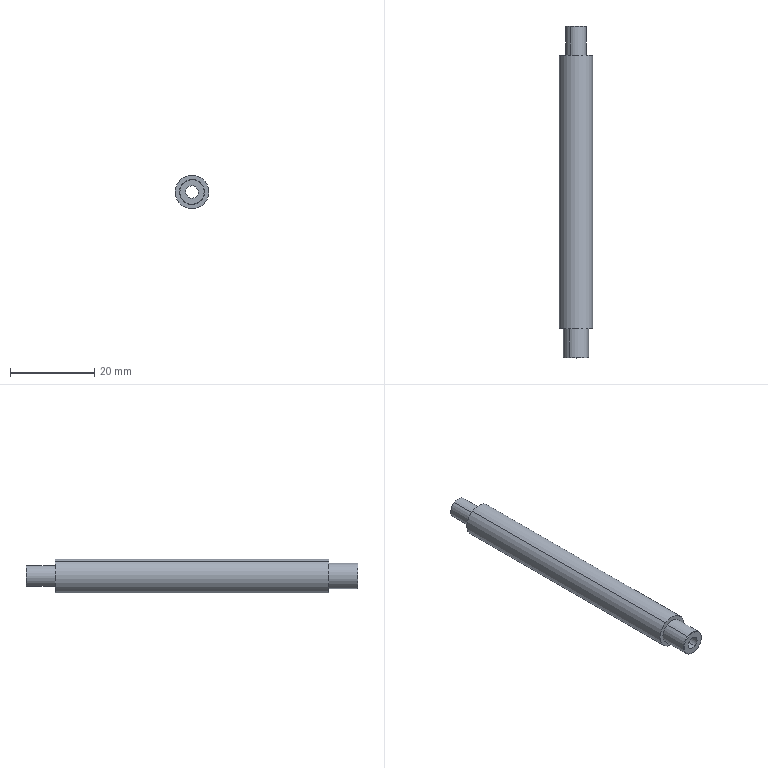Component | SolidWorks | WireFeedingTube-1 | 1 solid | 16 faces | box 8 x 79 x 8 mm | volume 3044 mm3 | cylinder 8 | cone 4 | plane 4 | commonest cylinder face diameters 6 x2 8 x2 5 x2 3 x2
build123d program:
from build123d import *

# Parameters (mm, degrees)
CHAMFER1_SIZE = 0.1


with BuildPart() as part:
    # Sketch1 → Revolve1 (revolve)
    with BuildSketch(Plane(origin=(0, 0, 0), x_dir=(0, 0, -1), z_dir=(1, 0, 0)), mode=Mode.PRIVATE) as revolve1_sk:
        Polygon((-13.875, 1.5), (65.125, 1.5), (65.125, 2.5), (58.125, 2.5), (58.125, 4), (-6.875, 4), (-6.875, 3), (-13.875, 3), align=None)
    revolve(revolve1_sk.sketch.rotate(Axis((0, 0, 14.85), (0, 0, -1)), 90), axis=Axis((0, 0, 14.85), (0, 0, -1)))

    # Chamfer1
    chamfer1_edges = [part.edges().sort_by_distance(p)[0] for p in [
        (-3, 0, 13.875),
        (-2.5, 0, -65.125),
    ]]
    chamfer(chamfer1_edges, length=CHAMFER1_SIZE)


solid = part.part

# Placed as in the assembly
solid = solid.moved(Location((37.32, 27.381, 185), (90, 0, 0)))
STEP:
#1=CARTESIAN_POINT('',(1.419,3.642,7.363));
#2=VERTEX_POINT('',#1);
#3=CARTESIAN_POINT('',(1.52,3.642,7.204));
#4=VERTEX_POINT('',#3);
#5=CARTESIAN_POINT('',(1.469,3.642,7.283));
#6=DIRECTION('',(0.,1.,-0.));
#7=DIRECTION('',(0.5343,0.,-0.8453));
#8=AXIS2_PLACEMENT_3D('',#5,#6,#7);
#9=CIRCLE('',#8,0.09449);
#10=EDGE_CURVE('',#2,#4,#9,.T.);
#11=ORIENTED_EDGE('',*,*,#10,.F.);
#12=CARTESIAN_POINT('',(1.417,3.638,7.367));
#13=VERTEX_POINT('',#12);
#14=CARTESIAN_POINT('',(1.417,3.638,7.367));
#15=DIRECTION('',(-0.3778,-0.7071,0.5977));
#16=VECTOR('',#15,39.37);
#17=LINE('',#14,#16);
#18=EDGE_CURVE('',#2,#13,#17,.T.);
#19=ORIENTED_EDGE('',*,*,#18,.T.);
#20=CARTESIAN_POINT('',(1.522,3.638,7.2));
#21=VERTEX_POINT('',#20);
#22=CARTESIAN_POINT('',(1.469,3.638,7.283));
#23=DIRECTION('',(-0.,-1.,0.));
#24=DIRECTION('',(0.5343,0.,-0.8453));
#25=AXIS2_PLACEMENT_3D('',#22,#23,#24);
#26=CIRCLE('',#25,0.09843);
#27=EDGE_CURVE('',#21,#13,#26,.T.);
#28=ORIENTED_EDGE('',*,*,#27,.F.);
#29=CARTESIAN_POINT('',(1.522,3.638,7.2));
#30=DIRECTION('',(0.3778,-0.7071,-0.5977));
#31=VECTOR('',#30,39.37);
#32=LINE('',#29,#31);
#33=EDGE_CURVE('',#4,#21,#32,.T.);
#34=ORIENTED_EDGE('',*,*,#33,.F.);
#35=EDGE_LOOP('',(#11,#19,#28,#34));
#36=FACE_OUTER_BOUND('',#35,.T.);
#37=CARTESIAN_POINT('',(1.469,3.638,7.283));
#38=DIRECTION('',(-0.,-1.,0.));
#39=DIRECTION('',(0.5343,0.,-0.8453));
#40=AXIS2_PLACEMENT_3D('',#37,#38,#39);
#41=CONICAL_SURFACE('',#40,0.09843,0.7854);
#42=ADVANCED_FACE('',(#36),#41,.T.);
#43=CARTESIAN_POINT('',(1.53,0.5317,7.187));
#44=VERTEX_POINT('',#43);
#45=CARTESIAN_POINT('',(1.408,0.5317,7.38));
#46=VERTEX_POINT('',#45);
#47=CARTESIAN_POINT('',(1.469,0.5317,7.283));
#48=DIRECTION('',(-0.,-1.,0.));
#49=DIRECTION('',(-0.5343,0.,0.8453));
#50=AXIS2_PLACEMENT_3D('',#47,#48,#49);
#51=CIRCLE('',#50,0.1142);
#52=EDGE_CURVE('',#44,#46,#51,.T.);
#53=ORIENTED_EDGE('',*,*,#52,.F.);
#54=CARTESIAN_POINT('',(1.532,0.5357,7.184));
#55=VERTEX_POINT('',#54);
#56=CARTESIAN_POINT('',(1.53,0.5317,7.187));
#57=DIRECTION('',(0.3778,0.7071,-0.5977));
#58=VECTOR('',#57,39.37);
#59=LINE('',#56,#58);
#60=EDGE_CURVE('',#44,#55,#59,.T.);
#61=ORIENTED_EDGE('',*,*,#60,.T.);
#62=CARTESIAN_POINT('',(1.406,0.5357,7.383));
#63=VERTEX_POINT('',#62);
#64=CARTESIAN_POINT('',(1.469,0.5357,7.283));
#65=DIRECTION('',(0.,1.,-0.));
#66=DIRECTION('',(-0.5343,0.,0.8453));
#67=AXIS2_PLACEMENT_3D('',#64,#65,#66);
#68=CIRCLE('',#67,0.1181);
#69=EDGE_CURVE('',#63,#55,#68,.T.);
#70=ORIENTED_EDGE('',*,*,#69,.F.);
#71=CARTESIAN_POINT('',(1.408,0.5317,7.38));
#72=DIRECTION('',(-0.3778,0.7071,0.5977));
#73=VECTOR('',#72,39.37);
#74=LINE('',#71,#73);
#75=EDGE_CURVE('',#46,#63,#74,.T.);
#76=ORIENTED_EDGE('',*,*,#75,.F.);
#77=EDGE_LOOP('',(#53,#61,#70,#76));
#78=FACE_OUTER_BOUND('',#77,.T.);
#79=CARTESIAN_POINT('',(1.469,0.5317,7.283));
#80=DIRECTION('',(0.,1.,-0.));
#81=DIRECTION('',(-0.5343,0.,0.8453));
#82=AXIS2_PLACEMENT_3D('',#79,#80,#81);
#83=CONICAL_SURFACE('',#82,0.1142,0.7854);
#84=ADVANCED_FACE('',(#78),#83,.T.);
#85=CARTESIAN_POINT('',(1.532,0.8073,7.184));
#86=VERTEX_POINT('',#85);
#87=CARTESIAN_POINT('',(1.406,0.8073,7.383));
#88=VERTEX_POINT('',#87);
#89=CARTESIAN_POINT('',(1.469,0.8073,7.283));
#90=DIRECTION('',(-0.,-1.,0.));
#91=DIRECTION('',(0.5343,0.,-0.8453));
#92=AXIS2_PLACEMENT_3D('',#89,#90,#91);
#93=CIRCLE('',#92,0.1181);
#94=EDGE_CURVE('',#86,#88,#93,.T.);
#95=ORIENTED_EDGE('',*,*,#94,.T.);
#96=CARTESIAN_POINT('',(1.406,0.4934,7.383));
#97=DIRECTION('',(-0.,-1.,0.));
#98=VECTOR('',#97,39.37);
#99=LINE('',#96,#98);
#100=EDGE_CURVE('',#88,#63,#99,.T.);
#101=ORIENTED_EDGE('',*,*,#100,.T.);
#102=ORIENTED_EDGE('',*,*,#69,.T.);
#103=CARTESIAN_POINT('',(1.532,0.4934,7.184));
#104=DIRECTION('',(-0.,-1.,0.));
#105=VECTOR('',#104,39.37);
#106=LINE('',#103,#105);
#107=EDGE_CURVE('',#86,#55,#106,.T.);
#108=ORIENTED_EDGE('',*,*,#107,.F.);
#109=EDGE_LOOP('',(#95,#101,#102,#108));
#110=FACE_OUTER_BOUND('',#109,.T.);
#111=CARTESIAN_POINT('',(1.469,0.4934,7.283));
#112=DIRECTION('',(-0.,-1.,0.));
#113=DIRECTION('',(0.5343,0.,-0.8453));
#114=AXIS2_PLACEMENT_3D('',#111,#112,#113);
#115=CYLINDRICAL_SURFACE('',#114,0.1181);
#116=ADVANCED_FACE('',(#110),#115,.T.);
#117=CARTESIAN_POINT('',(1.553,3.366,7.15));
#118=VERTEX_POINT('',#117);
#119=CARTESIAN_POINT('',(1.385,3.366,7.417));
#120=VERTEX_POINT('',#119);
#121=CARTESIAN_POINT('',(1.469,3.366,7.283));
#122=DIRECTION('',(-0.,-1.,0.));
#123=DIRECTION('',(0.5343,0.,-0.8453));
#124=AXIS2_PLACEMENT_3D('',#121,#122,#123);
#125=CIRCLE('',#124,0.1575);
#126=EDGE_CURVE('',#118,#120,#125,.T.);
#127=ORIENTED_EDGE('',*,*,#126,.T.);
#128=CARTESIAN_POINT('',(1.385,0.8073,7.417));
#129=VERTEX_POINT('',#128);
#130=CARTESIAN_POINT('',(1.385,0.4934,7.417));
#131=DIRECTION('',(-0.,-1.,0.));
#132=VECTOR('',#131,39.37);
#133=LINE('',#130,#132);
#134=EDGE_CURVE('',#120,#129,#133,.T.);
#135=ORIENTED_EDGE('',*,*,#134,.T.);
#136=CARTESIAN_POINT('',(1.553,0.8073,7.15));
#137=VERTEX_POINT('',#136);
#138=CARTESIAN_POINT('',(1.469,0.8073,7.283));
#139=DIRECTION('',(-0.,-1.,0.));
#140=DIRECTION('',(0.5343,0.,-0.8453));
#141=AXIS2_PLACEMENT_3D('',#138,#139,#140);
#142=CIRCLE('',#141,0.1575);
#143=EDGE_CURVE('',#137,#129,#142,.T.);
#144=ORIENTED_EDGE('',*,*,#143,.F.);
#145=CARTESIAN_POINT('',(1.553,0.4934,7.15));
#146=DIRECTION('',(-0.,-1.,0.));
#147=VECTOR('',#146,39.37);
#148=LINE('',#145,#147);
#149=EDGE_CURVE('',#118,#137,#148,.T.);
#150=ORIENTED_EDGE('',*,*,#149,.F.);
#151=EDGE_LOOP('',(#127,#135,#144,#150));
#152=FACE_OUTER_BOUND('',#151,.T.);
#153=CARTESIAN_POINT('',(1.469,0.4934,7.283));
#154=DIRECTION('',(-0.,-1.,0.));
#155=DIRECTION('',(0.5343,0.,-0.8453));
#156=AXIS2_PLACEMENT_3D('',#153,#154,#155);
#157=CYLINDRICAL_SURFACE('',#156,0.1575);
#158=ADVANCED_FACE('',(#152),#157,.T.);
#159=ORIENTED_EDGE('',*,*,#27,.T.);
#160=CARTESIAN_POINT('',(1.417,3.366,7.367));
#161=VERTEX_POINT('',#160);
#162=CARTESIAN_POINT('',(1.417,0.4934,7.367));
#163=DIRECTION('',(-0.,-1.,0.));
#164=VECTOR('',#163,39.37);
#165=LINE('',#162,#164);
#166=EDGE_CURVE('',#13,#161,#165,.T.);
#167=ORIENTED_EDGE('',*,*,#166,.T.);
#168=CARTESIAN_POINT('',(1.522,3.366,7.2));
#169=VERTEX_POINT('',#168);
#170=CARTESIAN_POINT('',(1.469,3.366,7.283));
#171=DIRECTION('',(-0.,-1.,0.));
#172=DIRECTION('',(0.5343,0.,-0.8453));
#173=AXIS2_PLACEMENT_3D('',#170,#171,#172);
#174=CIRCLE('',#173,0.09843);
#175=EDGE_CURVE('',#169,#161,#174,.T.);
#176=ORIENTED_EDGE('',*,*,#175,.F.);
#177=CARTESIAN_POINT('',(1.522,0.4934,7.2));
#178=DIRECTION('',(-0.,-1.,0.));
#179=VECTOR('',#178,39.37);
#180=LINE('',#177,#179);
#181=EDGE_CURVE('',#21,#169,#180,.T.);
#182=ORIENTED_EDGE('',*,*,#181,.F.);
#183=EDGE_LOOP('',(#159,#167,#176,#182));
#184=FACE_OUTER_BOUND('',#183,.T.);
#185=CARTESIAN_POINT('',(1.469,0.4934,7.283));
#186=DIRECTION('',(-0.,-1.,0.));
#187=DIRECTION('',(0.5343,0.,-0.8453));
#188=AXIS2_PLACEMENT_3D('',#185,#186,#187);
#189=CYLINDRICAL_SURFACE('',#188,0.09843);
#190=ADVANCED_FACE('',(#184),#189,.T.);
#191=CARTESIAN_POINT('',(1.438,3.642,7.333));
#192=VERTEX_POINT('',#191);
#193=CARTESIAN_POINT('',(1.501,3.642,7.234));
#194=VERTEX_POINT('',#193);
#195=CARTESIAN_POINT('',(1.469,3.642,7.283));
#196=DIRECTION('',(-0.,-1.,0.));
#197=DIRECTION('',(0.5343,0.,-0.8453));
#198=AXIS2_PLACEMENT_3D('',#195,#196,#197);
#199=CIRCLE('',#198,0.05906);
#200=EDGE_CURVE('',#192,#194,#199,.T.);
#201=ORIENTED_EDGE('',*,*,#200,.F.);
#202=CARTESIAN_POINT('',(1.438,0.5317,7.333));
#203=VERTEX_POINT('',#202);
#204=CARTESIAN_POINT('',(1.438,0.4934,7.333));
#205=DIRECTION('',(-0.,-1.,0.));
#206=VECTOR('',#205,39.37);
#207=LINE('',#204,#206);
#208=EDGE_CURVE('',#192,#203,#207,.T.);
#209=ORIENTED_EDGE('',*,*,#208,.T.);
#210=CARTESIAN_POINT('',(1.501,0.5317,7.234));
#211=VERTEX_POINT('',#210);
#212=CARTESIAN_POINT('',(1.469,0.5317,7.283));
#213=DIRECTION('',(-0.,-1.,0.));
#214=DIRECTION('',(0.5343,0.,-0.8453));
#215=AXIS2_PLACEMENT_3D('',#212,#213,#214);
#216=CIRCLE('',#215,0.05906);
#217=EDGE_CURVE('',#203,#211,#216,.T.);
#218=ORIENTED_EDGE('',*,*,#217,.T.);
#219=CARTESIAN_POINT('',(1.501,0.4934,7.234));
#220=DIRECTION('',(-0.,-1.,0.));
#221=VECTOR('',#220,39.37);
#222=LINE('',#219,#221);
#223=EDGE_CURVE('',#194,#211,#222,.T.);
#224=ORIENTED_EDGE('',*,*,#223,.F.);
#225=EDGE_LOOP('',(#201,#209,#218,#224));
#226=FACE_OUTER_BOUND('',#225,.T.);
#227=CARTESIAN_POINT('',(1.469,0.4934,7.283));
#228=DIRECTION('',(-0.,-1.,0.));
#229=DIRECTION('',(0.5343,0.,-0.8453));
#230=AXIS2_PLACEMENT_3D('',#227,#228,#229);
#231=CYLINDRICAL_SURFACE('',#230,0.05906);
#232=ADVANCED_FACE('',(#226),#231,.F.);
#233=CARTESIAN_POINT('',(1.469,0.5317,7.283));
#234=DIRECTION('',(-0.,-1.,0.));
#235=DIRECTION('',(-0.5343,0.,0.8453));
#236=AXIS2_PLACEMENT_3D('',#233,#234,#235);
#237=CIRCLE('',#236,0.1142);
#238=EDGE_CURVE('',#46,#44,#237,.T.);
#239=ORIENTED_EDGE('',*,*,#238,.T.);
#240=ORIENTED_EDGE('',*,*,#52,.T.);
#241=EDGE_LOOP('',(#239,#240));
#242=FACE_OUTER_BOUND('',#241,.T.);
#243=CARTESIAN_POINT('',(1.469,0.5317,7.283));
#244=DIRECTION('',(-0.,-1.,0.));
#245=DIRECTION('',(0.5343,0.,-0.8453));
#246=AXIS2_PLACEMENT_3D('',#243,#244,#245);
#247=CIRCLE('',#246,0.05906);
#248=EDGE_CURVE('',#211,#203,#247,.T.);
#249=ORIENTED_EDGE('',*,*,#248,.F.);
#250=ORIENTED_EDGE('',*,*,#217,.F.);
#251=EDGE_LOOP('',(#249,#250));
#252=FACE_BOUND('',#251,.T.);
#253=CARTESIAN_POINT('',(1.569,0.5317,7.347));
#254=DIRECTION('',(0.,1.,-0.));
#255=DIRECTION('',(-0.5343,0.,0.8453));
#256=AXIS2_PLACEMENT_3D('',#253,#254,#255);
#257=PLANE('',#256);
#258=ADVANCED_FACE('',(#242,#252),#257,.F.);
#259=ORIENTED_EDGE('',*,*,#208,.F.);
#260=CARTESIAN_POINT('',(1.469,3.642,7.283));
#261=DIRECTION('',(-0.,-1.,0.));
#262=DIRECTION('',(0.5343,0.,-0.8453));
#263=AXIS2_PLACEMENT_3D('',#260,#261,#262);
#264=CIRCLE('',#263,0.05906);
#265=EDGE_CURVE('',#194,#192,#264,.T.);
#266=ORIENTED_EDGE('',*,*,#265,.F.);
#267=ORIENTED_EDGE('',*,*,#223,.T.);
#268=ORIENTED_EDGE('',*,*,#248,.T.);
#269=EDGE_LOOP('',(#259,#266,#267,#268));
#270=FACE_OUTER_BOUND('',#269,.T.);
#271=CARTESIAN_POINT('',(1.469,0.4934,7.283));
#272=DIRECTION('',(-0.,-1.,0.));
#273=DIRECTION('',(0.5343,0.,-0.8453));
#274=AXIS2_PLACEMENT_3D('',#271,#272,#273);
#275=CYLINDRICAL_SURFACE('',#274,0.05906);
#276=ADVANCED_FACE('',(#270),#275,.F.);
#277=CARTESIAN_POINT('',(1.469,3.642,7.283));
#278=DIRECTION('',(0.,1.,-0.));
#279=DIRECTION('',(0.5343,0.,-0.8453));
#280=AXIS2_PLACEMENT_3D('',#277,#278,#279);
#281=CIRCLE('',#280,0.09449);
#282=EDGE_CURVE('',#4,#2,#281,.T.);
#283=ORIENTED_EDGE('',*,*,#282,.T.);
#284=ORIENTED_EDGE('',*,*,#10,.T.);
#285=EDGE_LOOP('',(#283,#284));
#286=FACE_OUTER_BOUND('',#285,.T.);
#287=ORIENTED_EDGE('',*,*,#265,.T.);
#288=ORIENTED_EDGE('',*,*,#200,.T.);
#289=EDGE_LOOP('',(#287,#288));
#290=FACE_BOUND('',#289,.T.);
#291=CARTESIAN_POINT('',(1.519,3.642,7.315));
#292=DIRECTION('',(-0.,-1.,0.));
#293=DIRECTION('',(0.5343,-0.,-0.8453));
#294=AXIS2_PLACEMENT_3D('',#291,#292,#293);
#295=PLANE('',#294);
#296=ADVANCED_FACE('',(#286,#290),#295,.F.);
#297=ORIENTED_EDGE('',*,*,#166,.F.);
#298=CARTESIAN_POINT('',(1.469,3.638,7.283));
#299=DIRECTION('',(-0.,-1.,0.));
#300=DIRECTION('',(0.5343,0.,-0.8453));
#301=AXIS2_PLACEMENT_3D('',#298,#299,#300);
#302=CIRCLE('',#301,0.09843);
#303=EDGE_CURVE('',#13,#21,#302,.T.);
#304=ORIENTED_EDGE('',*,*,#303,.T.);
#305=ORIENTED_EDGE('',*,*,#181,.T.);
#306=CARTESIAN_POINT('',(1.469,3.366,7.283));
#307=DIRECTION('',(-0.,-1.,0.));
#308=DIRECTION('',(0.5343,0.,-0.8453));
#309=AXIS2_PLACEMENT_3D('',#306,#307,#308);
#310=CIRCLE('',#309,0.09843);
#311=EDGE_CURVE('',#161,#169,#310,.T.);
#312=ORIENTED_EDGE('',*,*,#311,.F.);
#313=EDGE_LOOP('',(#297,#304,#305,#312));
#314=FACE_OUTER_BOUND('',#313,.T.);
#315=CARTESIAN_POINT('',(1.469,0.4934,7.283));
#316=DIRECTION('',(-0.,-1.,0.));
#317=DIRECTION('',(0.5343,0.,-0.8453));
#318=AXIS2_PLACEMENT_3D('',#315,#316,#317);
#319=CYLINDRICAL_SURFACE('',#318,0.09843);
#320=ADVANCED_FACE('',(#314),#319,.T.);
#321=ORIENTED_EDGE('',*,*,#126,.F.);
#322=CARTESIAN_POINT('',(1.469,3.366,7.283));
#323=DIRECTION('',(-0.,-1.,0.));
#324=DIRECTION('',(0.5343,0.,-0.8453));
#325=AXIS2_PLACEMENT_3D('',#322,#323,#324);
#326=CIRCLE('',#325,0.1575);
#327=EDGE_CURVE('',#120,#118,#326,.T.);
#328=ORIENTED_EDGE('',*,*,#327,.F.);
#329=EDGE_LOOP('',(#321,#328));
#330=FACE_OUTER_BOUND('',#329,.T.);
#331=ORIENTED_EDGE('',*,*,#175,.T.);
#332=ORIENTED_EDGE('',*,*,#311,.T.);
#333=EDGE_LOOP('',(#331,#332));
#334=FACE_BOUND('',#333,.T.);
#335=CARTESIAN_POINT('',(1.553,3.366,7.336));
#336=DIRECTION('',(-0.,-1.,0.));
#337=DIRECTION('',(0.5343,-0.,-0.8453));
#338=AXIS2_PLACEMENT_3D('',#335,#336,#337);
#339=PLANE('',#338);
#340=ADVANCED_FACE('',(#330,#334),#339,.F.);
#341=ORIENTED_EDGE('',*,*,#134,.F.);
#342=ORIENTED_EDGE('',*,*,#327,.T.);
#343=ORIENTED_EDGE('',*,*,#149,.T.);
#344=CARTESIAN_POINT('',(1.469,0.8073,7.283));
#345=DIRECTION('',(-0.,-1.,0.));
#346=DIRECTION('',(0.5343,0.,-0.8453));
#347=AXIS2_PLACEMENT_3D('',#344,#345,#346);
#348=CIRCLE('',#347,0.1575);
#349=EDGE_CURVE('',#129,#137,#348,.T.);
#350=ORIENTED_EDGE('',*,*,#349,.F.);
#351=EDGE_LOOP('',(#341,#342,#343,#350));
#352=FACE_OUTER_BOUND('',#351,.T.);
#353=CARTESIAN_POINT('',(1.469,0.4934,7.283));
#354=DIRECTION('',(-0.,-1.,0.));
#355=DIRECTION('',(0.5343,0.,-0.8453));
#356=AXIS2_PLACEMENT_3D('',#353,#354,#355);
#357=CYLINDRICAL_SURFACE('',#356,0.1575);
#358=ADVANCED_FACE('',(#352),#357,.T.);
#359=ORIENTED_EDGE('',*,*,#94,.F.);
#360=CARTESIAN_POINT('',(1.469,0.8073,7.283));
#361=DIRECTION('',(-0.,-1.,0.));
#362=DIRECTION('',(0.5343,0.,-0.8453));
#363=AXIS2_PLACEMENT_3D('',#360,#361,#362);
#364=CIRCLE('',#363,0.1181);
#365=EDGE_CURVE('',#88,#86,#364,.T.);
#366=ORIENTED_EDGE('',*,*,#365,.F.);
#367=EDGE_LOOP('',(#359,#366));
#368=FACE_BOUND('',#367,.T.);
#369=ORIENTED_EDGE('',*,*,#143,.T.);
#370=ORIENTED_EDGE('',*,*,#349,.T.);
#371=EDGE_LOOP('',(#369,#370));
#372=FACE_OUTER_BOUND('',#371,.T.);
#373=CARTESIAN_POINT('',(1.602,0.8073,7.368));
#374=DIRECTION('',(0.,1.,-0.));
#375=DIRECTION('',(-0.5343,0.,0.8453));
#376=AXIS2_PLACEMENT_3D('',#373,#374,#375);
#377=PLANE('',#376);
#378=ADVANCED_FACE('',(#368,#372),#377,.F.);
#379=ORIENTED_EDGE('',*,*,#100,.F.);
#380=ORIENTED_EDGE('',*,*,#365,.T.);
#381=ORIENTED_EDGE('',*,*,#107,.T.);
#382=CARTESIAN_POINT('',(1.469,0.5357,7.283));
#383=DIRECTION('',(0.,1.,-0.));
#384=DIRECTION('',(-0.5343,0.,0.8453));
#385=AXIS2_PLACEMENT_3D('',#382,#383,#384);
#386=CIRCLE('',#385,0.1181);
#387=EDGE_CURVE('',#55,#63,#386,.T.);
#388=ORIENTED_EDGE('',*,*,#387,.T.);
#389=EDGE_LOOP('',(#379,#380,#381,#388));
#390=FACE_OUTER_BOUND('',#389,.T.);
#391=CARTESIAN_POINT('',(1.469,0.4934,7.283));
#392=DIRECTION('',(-0.,-1.,0.));
#393=DIRECTION('',(0.5343,0.,-0.8453));
#394=AXIS2_PLACEMENT_3D('',#391,#392,#393);
#395=CYLINDRICAL_SURFACE('',#394,0.1181);
#396=ADVANCED_FACE('',(#390),#395,.T.);
#397=ORIENTED_EDGE('',*,*,#60,.F.);
#398=ORIENTED_EDGE('',*,*,#238,.F.);
#399=ORIENTED_EDGE('',*,*,#75,.T.);
#400=ORIENTED_EDGE('',*,*,#387,.F.);
#401=EDGE_LOOP('',(#397,#398,#399,#400));
#402=FACE_OUTER_BOUND('',#401,.T.);
#403=CARTESIAN_POINT('',(1.469,0.5317,7.283));
#404=DIRECTION('',(0.,1.,-0.));
#405=DIRECTION('',(-0.5343,0.,0.8453));
#406=AXIS2_PLACEMENT_3D('',#403,#404,#405);
#407=CONICAL_SURFACE('',#406,0.1142,0.7854);
#408=ADVANCED_FACE('',(#402),#407,.T.);
#409=ORIENTED_EDGE('',*,*,#18,.F.);
#410=ORIENTED_EDGE('',*,*,#282,.F.);
#411=ORIENTED_EDGE('',*,*,#33,.T.);
#412=ORIENTED_EDGE('',*,*,#303,.F.);
#413=EDGE_LOOP('',(#409,#410,#411,#412));
#414=FACE_OUTER_BOUND('',#413,.T.);
#415=CARTESIAN_POINT('',(1.469,3.638,7.283));
#416=DIRECTION('',(-0.,-1.,0.));
#417=DIRECTION('',(0.5343,0.,-0.8453));
#418=AXIS2_PLACEMENT_3D('',#415,#416,#417);
#419=CONICAL_SURFACE('',#418,0.09843,0.7854);
#420=ADVANCED_FACE('',(#414),#419,.T.);
#421=CLOSED_SHELL('',(#42,#84,#116,#158,#190,#232,#258,#276,#296,#320,#340,#358,#378,#396,#408,#420));
#422=MANIFOLD_SOLID_BREP('',#421);
#423=CARTESIAN_POINT('',(0.,0.,0.));
#424=DIRECTION('',(0.,0.,1.));
#425=DIRECTION('',(1.,0.,0.));
#426=AXIS2_PLACEMENT_3D('',#423,#424,#425);
#427=(LENGTH_UNIT()NAMED_UNIT(*)SI_UNIT($,.METRE.));
#428=LENGTH_MEASURE_WITH_UNIT(LENGTH_MEASURE(0.0254),#427);
#429=DIMENSIONAL_EXPONENTS(1.,0.,0.,0.,0.,0.,0.);
#430=(CONVERSION_BASED_UNIT('',#428)LENGTH_UNIT()NAMED_UNIT(#429));
#431=UNCERTAINTY_MEASURE_WITH_UNIT(LENGTH_MEASURE(0.00001),#430,'','');
#432=(NAMED_UNIT(*)PLANE_ANGLE_UNIT()SI_UNIT($,.RADIAN.));
#433=(NAMED_UNIT(*)SI_UNIT($,.STERADIAN.)SOLID_ANGLE_UNIT());
#434=(GEOMETRIC_REPRESENTATION_CONTEXT(3)GLOBAL_UNCERTAINTY_ASSIGNED_CONTEXT((#431))GLOBAL_UNIT_ASSIGNED_CONTEXT((#430,#432,#433))REPRESENTATION_CONTEXT('',''));
#435=ADVANCED_BREP_SHAPE_REPRESENTATION('',(#422,#426),#434);
#436=COLOUR_RGB('',0.7922,0.8196,0.9333);
#437=FILL_AREA_STYLE_COLOUR('',#436);
#438=FILL_AREA_STYLE('',(#437));
#439=SURFACE_STYLE_FILL_AREA(#438);
#440=SURFACE_SIDE_STYLE('',(#439));
#441=SURFACE_STYLE_USAGE(.BOTH.,#440);
#442=PRESENTATION_STYLE_ASSIGNMENT((#441));
#443=STYLED_ITEM('',(#442),#422);
#444=(LENGTH_UNIT()NAMED_UNIT(*)SI_UNIT($,.METRE.));
#445=LENGTH_MEASURE_WITH_UNIT(LENGTH_MEASURE(0.0254),#444);
#446=DIMENSIONAL_EXPONENTS(1.,0.,0.,0.,0.,0.,0.);
#447=(CONVERSION_BASED_UNIT('',#445)LENGTH_UNIT()NAMED_UNIT(#446));
#448=UNCERTAINTY_MEASURE_WITH_UNIT(LENGTH_MEASURE(0.00001),#447,'','');
#449=(NAMED_UNIT(*)PLANE_ANGLE_UNIT()SI_UNIT($,.RADIAN.));
#450=(NAMED_UNIT(*)SI_UNIT($,.STERADIAN.)SOLID_ANGLE_UNIT());
#451=(GEOMETRIC_REPRESENTATION_CONTEXT(3)GLOBAL_UNCERTAINTY_ASSIGNED_CONTEXT((#448))GLOBAL_UNIT_ASSIGNED_CONTEXT((#447,#449,#450))REPRESENTATION_CONTEXT('',''));
#452=MECHANICAL_DESIGN_GEOMETRIC_PRESENTATION_REPRESENTATION('',(#443),#451);
#453=PRESENTATION_LAYER_ASSIGNMENT('','',(#443));